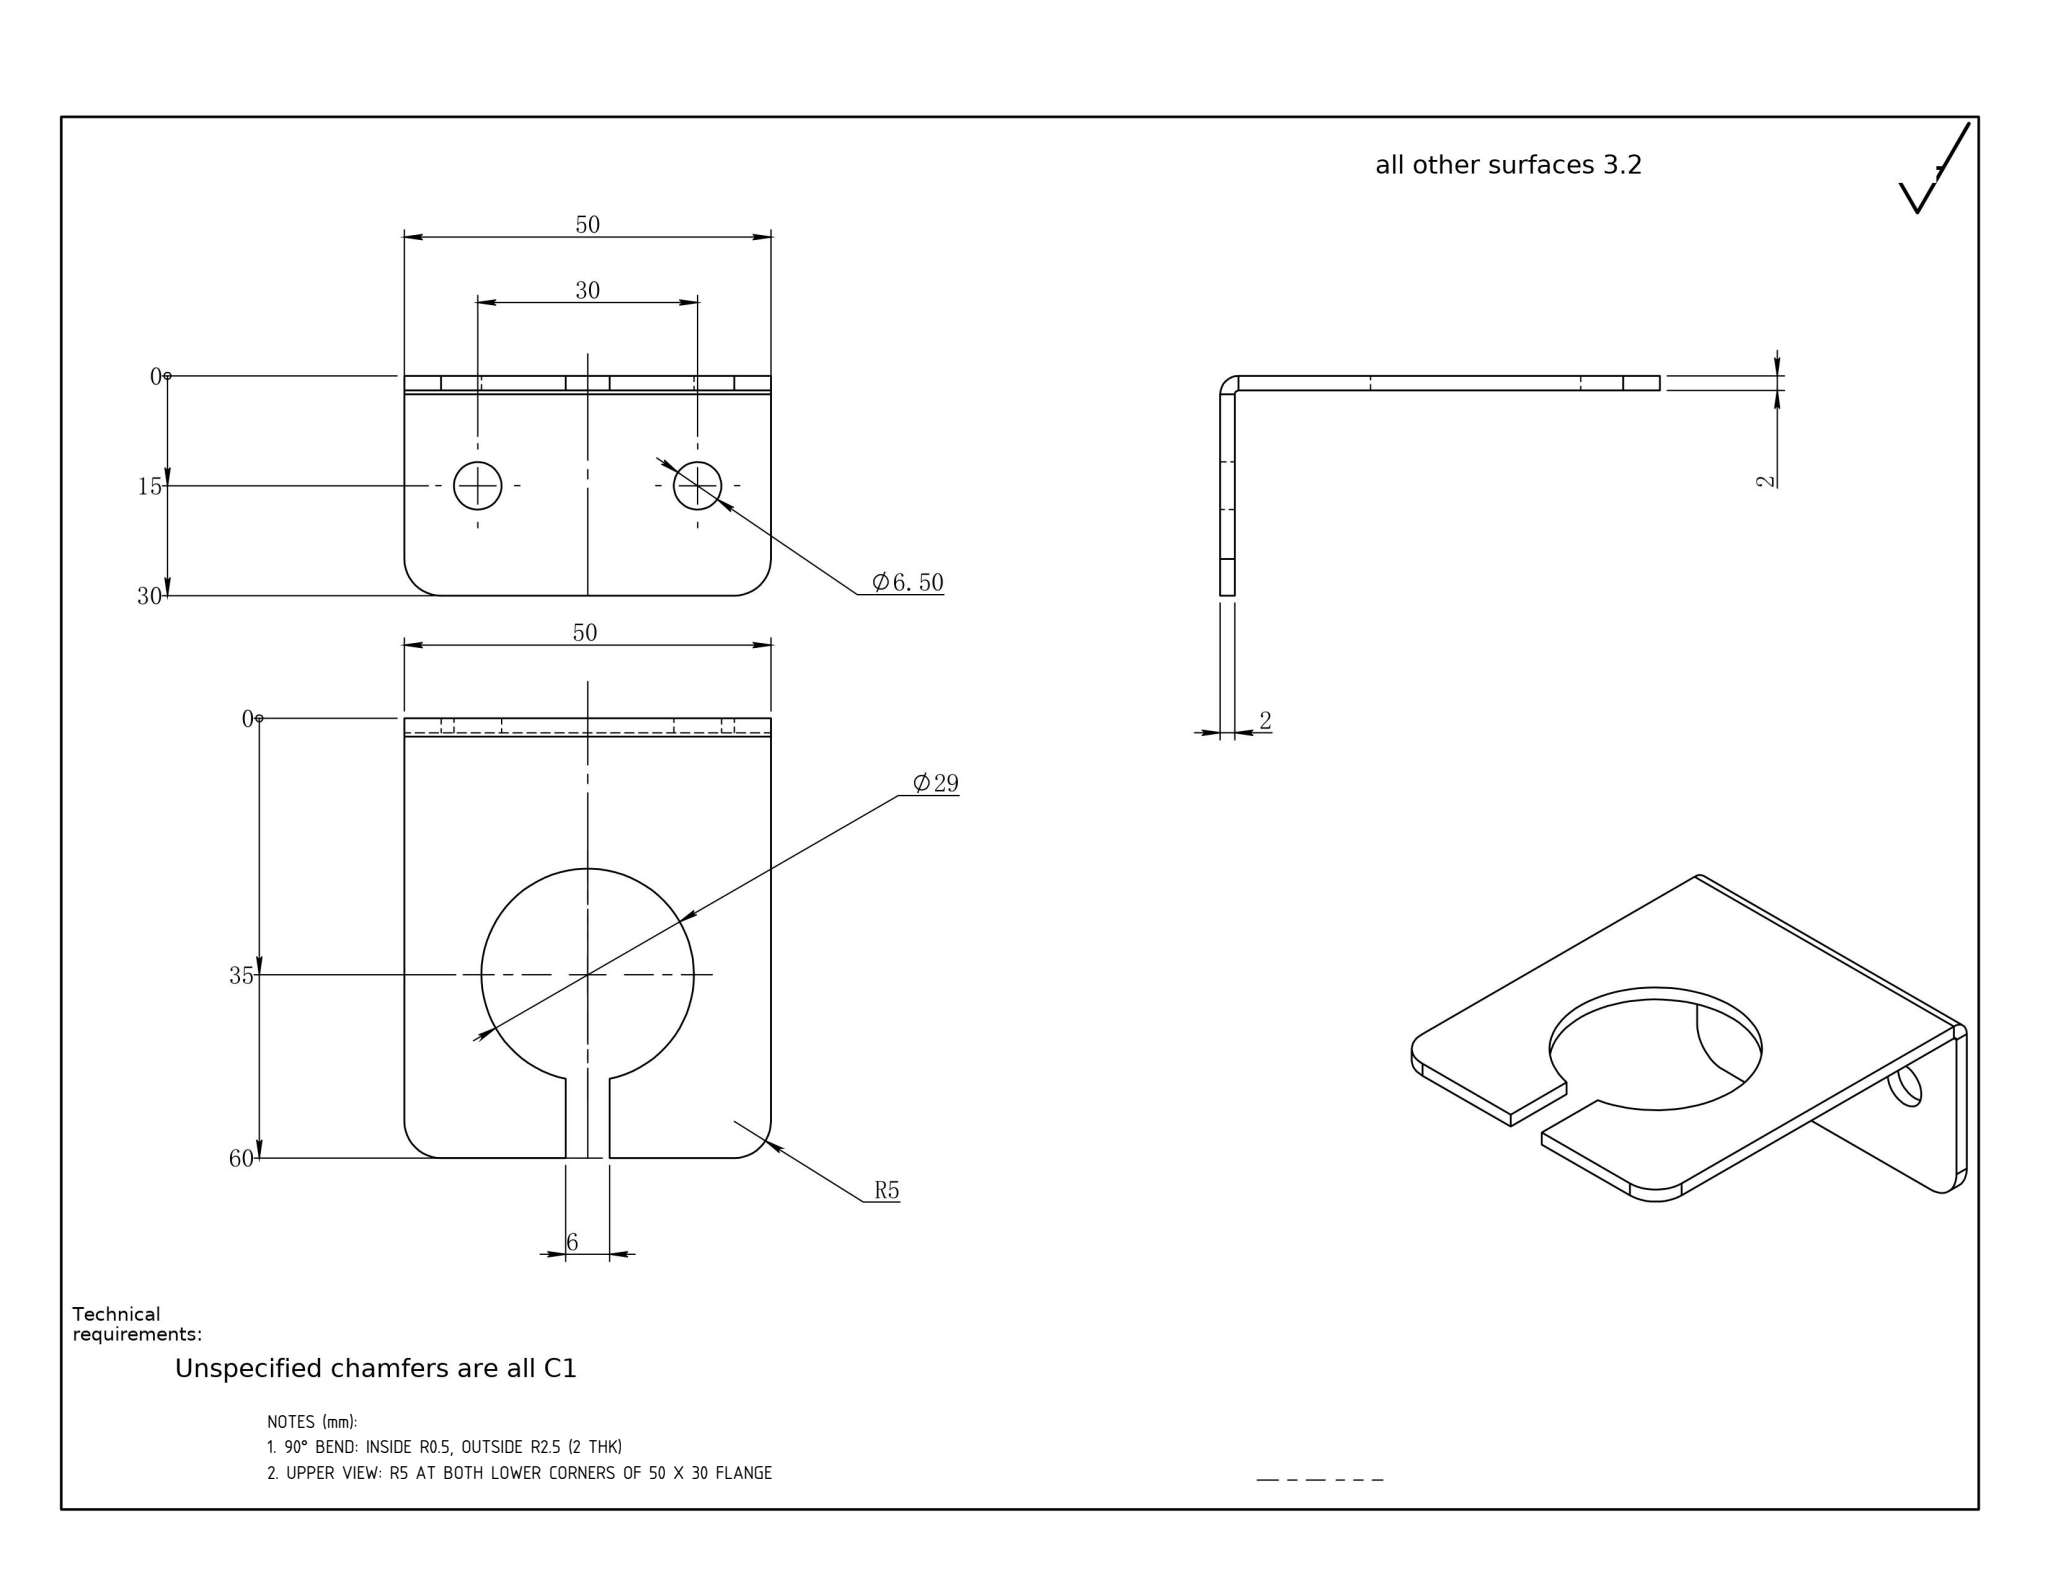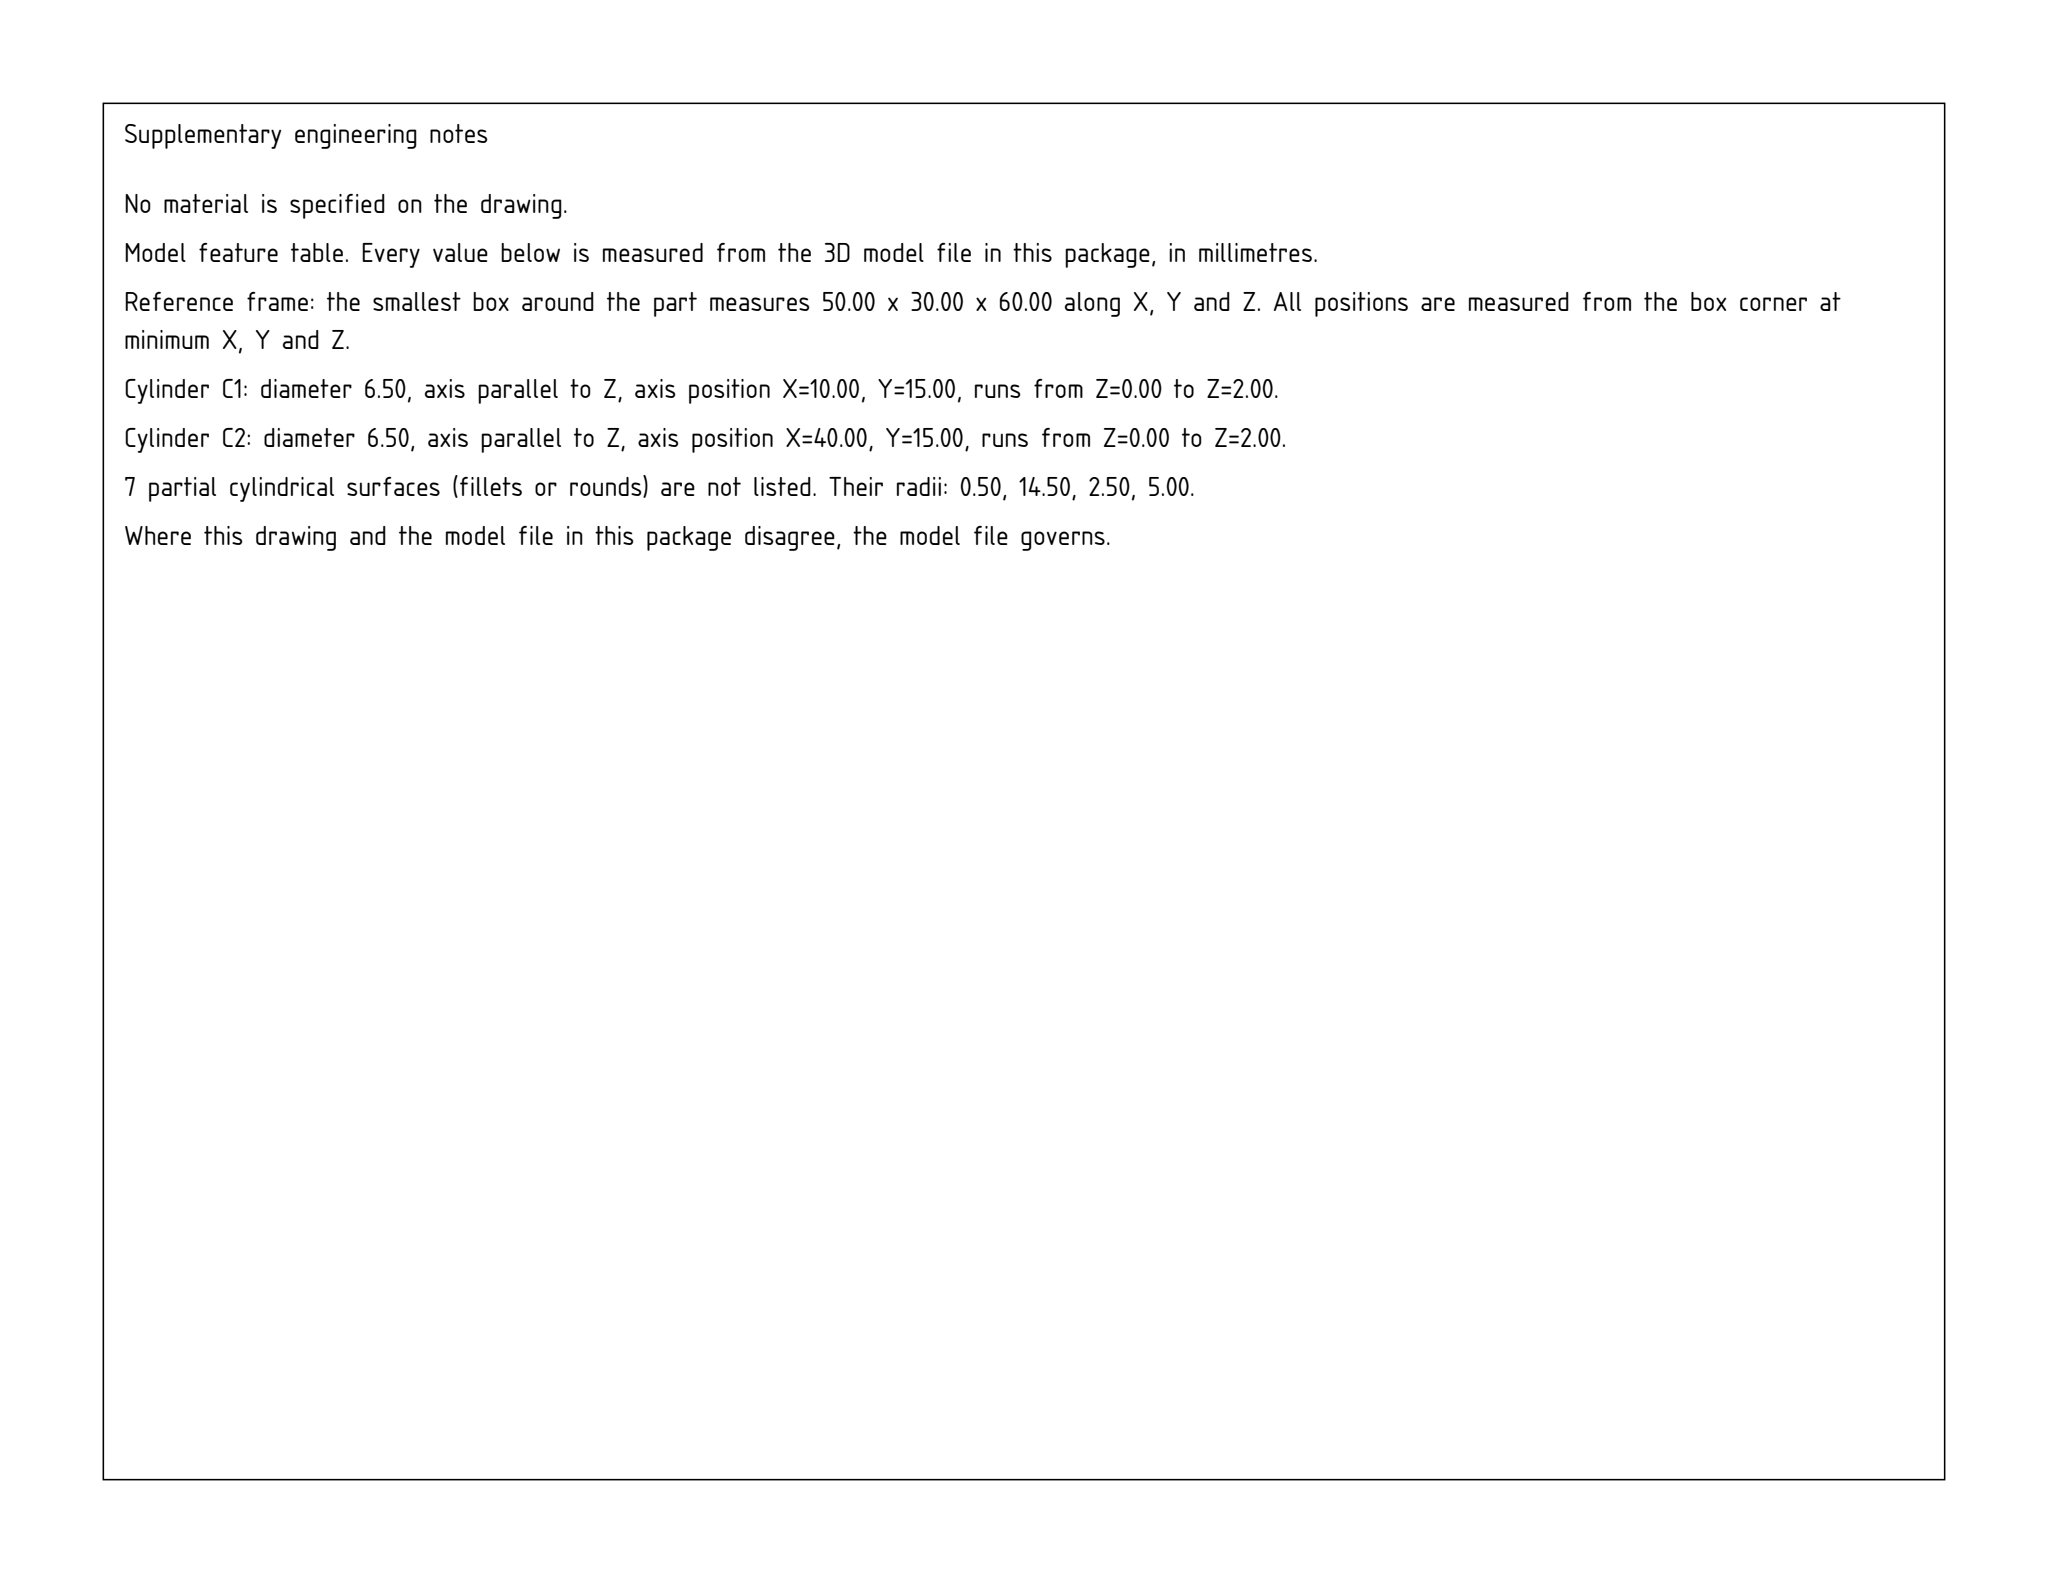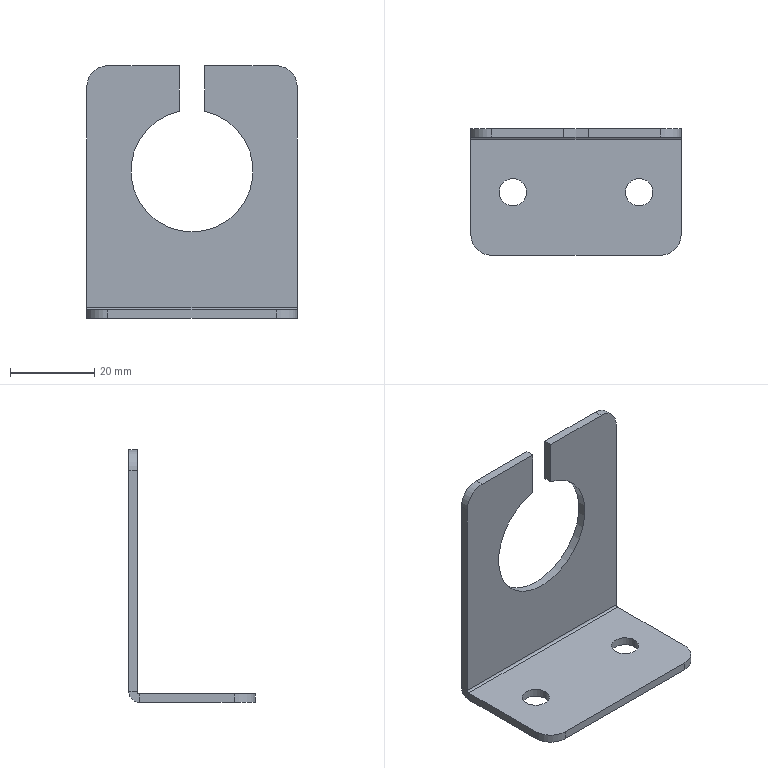Part | SolidWorks | mm | 1 solid | 26 faces | box 50 x 30 x 60 mm | volume 7112 mm3 | plane 15 | cylinder 11 | commonest cylinder face diameters 6.5 x4 10 x4 29 x1 5 x1 1 x1
Drawing notes:
90° BEND: INSIDE R0.5, OUTSIDE R2.5 (2 THK) | from the solid: cyl dia 1.0 & 5.0, axis x at y=27.5, z=2.5, len 50 = bend inner/outer radii with 2 wall
UPPER VIEW: R5 AT BOTH LOWER CORNERS OF 50 X 30 FLANGE | from the solid: Ø10 cyls, axis z, at (5,5) & (45,5), len 2 = R5 fillets on flange free edge (y=0 side), flange y 0-30, thk z 0-2
STEP:
#1=CARTESIAN_POINT('',(-18.25,-15.,-0.));
#2=VERTEX_POINT('',#1);
#3=CARTESIAN_POINT('',(-11.75,-15.,-0.));
#4=VERTEX_POINT('',#3);
#5=CARTESIAN_POINT('',(-15.,-15.,-0.));
#6=DIRECTION('',(0.,0.,1.));
#7=DIRECTION('',(1.,0.,0.));
#8=AXIS2_PLACEMENT_3D('',#5,#6,#7);
#9=CIRCLE('',#8,3.25);
#10=EDGE_CURVE('',#2,#4,#9,.T.);
#11=ORIENTED_EDGE('',*,*,#10,.F.);
#12=CARTESIAN_POINT('',(-18.25,-15.,2.));
#13=VERTEX_POINT('',#12);
#14=CARTESIAN_POINT('',(-18.25,-15.,2.));
#15=DIRECTION('',(0.,0.,1.));
#16=VECTOR('',#15,1000.);
#17=LINE('',#14,#16);
#18=EDGE_CURVE('',#2,#13,#17,.T.);
#19=ORIENTED_EDGE('',*,*,#18,.T.);
#20=CARTESIAN_POINT('',(-11.75,-15.,2.));
#21=VERTEX_POINT('',#20);
#22=CARTESIAN_POINT('',(-15.,-15.,2.));
#23=DIRECTION('',(0.,0.,1.));
#24=DIRECTION('',(1.,0.,0.));
#25=AXIS2_PLACEMENT_3D('',#22,#23,#24);
#26=CIRCLE('',#25,3.25);
#27=EDGE_CURVE('',#13,#21,#26,.T.);
#28=ORIENTED_EDGE('',*,*,#27,.T.);
#29=CARTESIAN_POINT('',(-11.75,-15.,2.));
#30=DIRECTION('',(0.,0.,1.));
#31=VECTOR('',#30,1000.);
#32=LINE('',#29,#31);
#33=EDGE_CURVE('',#4,#21,#32,.T.);
#34=ORIENTED_EDGE('',*,*,#33,.F.);
#35=EDGE_LOOP('',(#11,#19,#28,#34));
#36=FACE_OUTER_BOUND('',#35,.T.);
#37=CARTESIAN_POINT('',(-15.,-15.,2.));
#38=DIRECTION('',(0.,0.,1.));
#39=DIRECTION('',(1.,0.,0.));
#40=AXIS2_PLACEMENT_3D('',#37,#38,#39);
#41=CYLINDRICAL_SURFACE('',#40,3.25);
#42=ADVANCED_FACE('',(#36),#41,.F.);
#43=CARTESIAN_POINT('',(11.75,-15.,-0.));
#44=VERTEX_POINT('',#43);
#45=CARTESIAN_POINT('',(18.25,-15.,-0.));
#46=VERTEX_POINT('',#45);
#47=CARTESIAN_POINT('',(15.,-15.,-0.));
#48=DIRECTION('',(0.,0.,1.));
#49=DIRECTION('',(1.,0.,0.));
#50=AXIS2_PLACEMENT_3D('',#47,#48,#49);
#51=CIRCLE('',#50,3.25);
#52=EDGE_CURVE('',#44,#46,#51,.T.);
#53=ORIENTED_EDGE('',*,*,#52,.F.);
#54=CARTESIAN_POINT('',(11.75,-15.,2.));
#55=VERTEX_POINT('',#54);
#56=CARTESIAN_POINT('',(11.75,-15.,2.));
#57=DIRECTION('',(0.,0.,1.));
#58=VECTOR('',#57,1000.);
#59=LINE('',#56,#58);
#60=EDGE_CURVE('',#44,#55,#59,.T.);
#61=ORIENTED_EDGE('',*,*,#60,.T.);
#62=CARTESIAN_POINT('',(18.25,-15.,2.));
#63=VERTEX_POINT('',#62);
#64=CARTESIAN_POINT('',(15.,-15.,2.));
#65=DIRECTION('',(0.,0.,1.));
#66=DIRECTION('',(1.,0.,0.));
#67=AXIS2_PLACEMENT_3D('',#64,#65,#66);
#68=CIRCLE('',#67,3.25);
#69=EDGE_CURVE('',#55,#63,#68,.T.);
#70=ORIENTED_EDGE('',*,*,#69,.T.);
#71=CARTESIAN_POINT('',(18.25,-15.,2.));
#72=DIRECTION('',(0.,0.,1.));
#73=VECTOR('',#72,1000.);
#74=LINE('',#71,#73);
#75=EDGE_CURVE('',#46,#63,#74,.T.);
#76=ORIENTED_EDGE('',*,*,#75,.F.);
#77=EDGE_LOOP('',(#53,#61,#70,#76));
#78=FACE_OUTER_BOUND('',#77,.T.);
#79=CARTESIAN_POINT('',(15.,-15.,2.));
#80=DIRECTION('',(0.,0.,1.));
#81=DIRECTION('',(1.,0.,0.));
#82=AXIS2_PLACEMENT_3D('',#79,#80,#81);
#83=CYLINDRICAL_SURFACE('',#82,3.25);
#84=ADVANCED_FACE('',(#78),#83,.F.);
#85=CARTESIAN_POINT('',(3.,-0.,49.186));
#86=VERTEX_POINT('',#85);
#87=CARTESIAN_POINT('',(-3.,-0.,49.186));
#88=VERTEX_POINT('',#87);
#89=CARTESIAN_POINT('',(0.,-0.,35.));
#90=DIRECTION('',(0.,1.,0.));
#91=DIRECTION('',(0.,-0.,1.));
#92=AXIS2_PLACEMENT_3D('',#89,#90,#91);
#93=CIRCLE('',#92,14.5);
#94=EDGE_CURVE('',#86,#88,#93,.T.);
#95=ORIENTED_EDGE('',*,*,#94,.F.);
#96=CARTESIAN_POINT('',(3.,-0.,60.));
#97=VERTEX_POINT('',#96);
#98=CARTESIAN_POINT('',(3.,0.,0.));
#99=DIRECTION('',(0.,0.,-1.));
#100=VECTOR('',#99,1000.);
#101=LINE('',#98,#100);
#102=EDGE_CURVE('',#97,#86,#101,.T.);
#103=ORIENTED_EDGE('',*,*,#102,.F.);
#104=CARTESIAN_POINT('',(20.,-0.,60.));
#105=VERTEX_POINT('',#104);
#106=CARTESIAN_POINT('',(25.,-0.,60.));
#107=DIRECTION('',(-1.,0.,0.));
#108=VECTOR('',#107,1000.);
#109=LINE('',#106,#108);
#110=EDGE_CURVE('',#105,#97,#109,.T.);
#111=ORIENTED_EDGE('',*,*,#110,.F.);
#112=CARTESIAN_POINT('',(25.,-0.,55.));
#113=VERTEX_POINT('',#112);
#114=CARTESIAN_POINT('',(20.,-0.,55.));
#115=DIRECTION('',(0.,1.,0.));
#116=DIRECTION('',(0.,-0.,1.));
#117=AXIS2_PLACEMENT_3D('',#114,#115,#116);
#118=CIRCLE('',#117,5.);
#119=EDGE_CURVE('',#105,#113,#118,.T.);
#120=ORIENTED_EDGE('',*,*,#119,.T.);
#121=CARTESIAN_POINT('',(25.,-0.,2.5));
#122=VERTEX_POINT('',#121);
#123=CARTESIAN_POINT('',(25.,0.,0.));
#124=DIRECTION('',(0.,0.,-1.));
#125=VECTOR('',#124,1000.);
#126=LINE('',#123,#125);
#127=EDGE_CURVE('',#113,#122,#126,.T.);
#128=ORIENTED_EDGE('',*,*,#127,.T.);
#129=CARTESIAN_POINT('',(-25.,-0.,2.5));
#130=VERTEX_POINT('',#129);
#131=CARTESIAN_POINT('',(25.,-0.,2.5));
#132=DIRECTION('',(-1.,0.,0.));
#133=VECTOR('',#132,1000.);
#134=LINE('',#131,#133);
#135=EDGE_CURVE('',#122,#130,#134,.T.);
#136=ORIENTED_EDGE('',*,*,#135,.T.);
#137=CARTESIAN_POINT('',(-25.,-0.,55.));
#138=VERTEX_POINT('',#137);
#139=CARTESIAN_POINT('',(-25.,0.,0.));
#140=DIRECTION('',(0.,0.,-1.));
#141=VECTOR('',#140,1000.);
#142=LINE('',#139,#141);
#143=EDGE_CURVE('',#138,#130,#142,.T.);
#144=ORIENTED_EDGE('',*,*,#143,.F.);
#145=CARTESIAN_POINT('',(-20.,-0.,60.));
#146=VERTEX_POINT('',#145);
#147=CARTESIAN_POINT('',(-20.,-0.,55.));
#148=DIRECTION('',(0.,1.,0.));
#149=DIRECTION('',(0.,-0.,1.));
#150=AXIS2_PLACEMENT_3D('',#147,#148,#149);
#151=CIRCLE('',#150,5.);
#152=EDGE_CURVE('',#138,#146,#151,.T.);
#153=ORIENTED_EDGE('',*,*,#152,.T.);
#154=CARTESIAN_POINT('',(-3.,-0.,60.));
#155=VERTEX_POINT('',#154);
#156=CARTESIAN_POINT('',(25.,-0.,60.));
#157=DIRECTION('',(-1.,0.,0.));
#158=VECTOR('',#157,1000.);
#159=LINE('',#156,#158);
#160=EDGE_CURVE('',#155,#146,#159,.T.);
#161=ORIENTED_EDGE('',*,*,#160,.F.);
#162=CARTESIAN_POINT('',(-3.,0.,0.));
#163=DIRECTION('',(0.,-0.,1.));
#164=VECTOR('',#163,1000.);
#165=LINE('',#162,#164);
#166=EDGE_CURVE('',#88,#155,#165,.T.);
#167=ORIENTED_EDGE('',*,*,#166,.F.);
#168=EDGE_LOOP('',(#95,#103,#111,#120,#128,#136,#144,#153,#161,#167));
#169=FACE_OUTER_BOUND('',#168,.T.);
#170=CARTESIAN_POINT('',(25.,0.,0.));
#171=DIRECTION('',(0.,1.,0.));
#172=DIRECTION('',(0.,-0.,1.));
#173=AXIS2_PLACEMENT_3D('',#170,#171,#172);
#174=PLANE('',#173);
#175=ADVANCED_FACE('',(#169),#174,.T.);
#176=ORIENTED_EDGE('',*,*,#110,.T.);
#177=CARTESIAN_POINT('',(3.,-2.,60.));
#178=VERTEX_POINT('',#177);
#179=CARTESIAN_POINT('',(3.,-2.,60.));
#180=DIRECTION('',(0.,1.,0.));
#181=VECTOR('',#180,1000.);
#182=LINE('',#179,#181);
#183=EDGE_CURVE('',#178,#97,#182,.T.);
#184=ORIENTED_EDGE('',*,*,#183,.F.);
#185=CARTESIAN_POINT('',(20.,-2.,60.));
#186=VERTEX_POINT('',#185);
#187=CARTESIAN_POINT('',(25.,-2.,60.));
#188=DIRECTION('',(-1.,0.,0.));
#189=VECTOR('',#188,1000.);
#190=LINE('',#187,#189);
#191=EDGE_CURVE('',#186,#178,#190,.T.);
#192=ORIENTED_EDGE('',*,*,#191,.F.);
#193=CARTESIAN_POINT('',(20.,-2.,60.));
#194=DIRECTION('',(0.,1.,0.));
#195=VECTOR('',#194,1000.);
#196=LINE('',#193,#195);
#197=EDGE_CURVE('',#186,#105,#196,.T.);
#198=ORIENTED_EDGE('',*,*,#197,.T.);
#199=EDGE_LOOP('',(#176,#184,#192,#198));
#200=FACE_OUTER_BOUND('',#199,.T.);
#201=CARTESIAN_POINT('',(25.,-2.,60.));
#202=DIRECTION('',(0.,0.,1.));
#203=DIRECTION('',(1.,0.,0.));
#204=AXIS2_PLACEMENT_3D('',#201,#202,#203);
#205=PLANE('',#204);
#206=ADVANCED_FACE('',(#200),#205,.T.);
#207=CARTESIAN_POINT('',(-3.,-2.,60.));
#208=VERTEX_POINT('',#207);
#209=CARTESIAN_POINT('',(-20.,-2.,60.));
#210=VERTEX_POINT('',#209);
#211=CARTESIAN_POINT('',(25.,-2.,60.));
#212=DIRECTION('',(-1.,0.,0.));
#213=VECTOR('',#212,1000.);
#214=LINE('',#211,#213);
#215=EDGE_CURVE('',#208,#210,#214,.T.);
#216=ORIENTED_EDGE('',*,*,#215,.F.);
#217=CARTESIAN_POINT('',(-3.,-2.,60.));
#218=DIRECTION('',(0.,1.,0.));
#219=VECTOR('',#218,1000.);
#220=LINE('',#217,#219);
#221=EDGE_CURVE('',#208,#155,#220,.T.);
#222=ORIENTED_EDGE('',*,*,#221,.T.);
#223=ORIENTED_EDGE('',*,*,#160,.T.);
#224=CARTESIAN_POINT('',(-20.,-2.,60.));
#225=DIRECTION('',(0.,-1.,0.));
#226=VECTOR('',#225,1000.);
#227=LINE('',#224,#226);
#228=EDGE_CURVE('',#146,#210,#227,.T.);
#229=ORIENTED_EDGE('',*,*,#228,.T.);
#230=EDGE_LOOP('',(#216,#222,#223,#229));
#231=FACE_OUTER_BOUND('',#230,.T.);
#232=CARTESIAN_POINT('',(25.,-2.,60.));
#233=DIRECTION('',(0.,0.,1.));
#234=DIRECTION('',(1.,0.,0.));
#235=AXIS2_PLACEMENT_3D('',#232,#233,#234);
#236=PLANE('',#235);
#237=ADVANCED_FACE('',(#231),#236,.T.);
#238=CARTESIAN_POINT('',(3.,-2.,49.186));
#239=VERTEX_POINT('',#238);
#240=CARTESIAN_POINT('',(3.,-2.,-0.));
#241=DIRECTION('',(0.,0.,-1.));
#242=VECTOR('',#241,1000.);
#243=LINE('',#240,#242);
#244=EDGE_CURVE('',#178,#239,#243,.T.);
#245=ORIENTED_EDGE('',*,*,#244,.T.);
#246=CARTESIAN_POINT('',(-3.,-2.,49.186));
#247=VERTEX_POINT('',#246);
#248=CARTESIAN_POINT('',(0.,-2.,35.));
#249=DIRECTION('',(0.,1.,0.));
#250=DIRECTION('',(0.,-0.,1.));
#251=AXIS2_PLACEMENT_3D('',#248,#249,#250);
#252=CIRCLE('',#251,14.5);
#253=EDGE_CURVE('',#239,#247,#252,.T.);
#254=ORIENTED_EDGE('',*,*,#253,.T.);
#255=CARTESIAN_POINT('',(-3.,-2.,-0.));
#256=DIRECTION('',(0.,-0.,1.));
#257=VECTOR('',#256,1000.);
#258=LINE('',#255,#257);
#259=EDGE_CURVE('',#247,#208,#258,.T.);
#260=ORIENTED_EDGE('',*,*,#259,.T.);
#261=ORIENTED_EDGE('',*,*,#215,.T.);
#262=CARTESIAN_POINT('',(-25.,-2.,55.));
#263=VERTEX_POINT('',#262);
#264=CARTESIAN_POINT('',(-20.,-2.,55.));
#265=DIRECTION('',(0.,-1.,-0.));
#266=DIRECTION('',(0.,-0.,1.));
#267=AXIS2_PLACEMENT_3D('',#264,#265,#266);
#268=CIRCLE('',#267,5.);
#269=EDGE_CURVE('',#210,#263,#268,.T.);
#270=ORIENTED_EDGE('',*,*,#269,.T.);
#271=CARTESIAN_POINT('',(-25.,-2.,2.5));
#272=VERTEX_POINT('',#271);
#273=CARTESIAN_POINT('',(-25.,-2.,-0.));
#274=DIRECTION('',(0.,0.,-1.));
#275=VECTOR('',#274,1000.);
#276=LINE('',#273,#275);
#277=EDGE_CURVE('',#263,#272,#276,.T.);
#278=ORIENTED_EDGE('',*,*,#277,.T.);
#279=CARTESIAN_POINT('',(25.,-2.,2.5));
#280=VERTEX_POINT('',#279);
#281=CARTESIAN_POINT('',(25.,-2.,2.5));
#282=DIRECTION('',(-1.,0.,0.));
#283=VECTOR('',#282,1000.);
#284=LINE('',#281,#283);
#285=EDGE_CURVE('',#280,#272,#284,.T.);
#286=ORIENTED_EDGE('',*,*,#285,.F.);
#287=CARTESIAN_POINT('',(25.,-2.,55.));
#288=VERTEX_POINT('',#287);
#289=CARTESIAN_POINT('',(25.,-2.,-0.));
#290=DIRECTION('',(0.,0.,-1.));
#291=VECTOR('',#290,1000.);
#292=LINE('',#289,#291);
#293=EDGE_CURVE('',#288,#280,#292,.T.);
#294=ORIENTED_EDGE('',*,*,#293,.F.);
#295=CARTESIAN_POINT('',(20.,-2.,55.));
#296=DIRECTION('',(0.,-1.,-0.));
#297=DIRECTION('',(0.,-0.,1.));
#298=AXIS2_PLACEMENT_3D('',#295,#296,#297);
#299=CIRCLE('',#298,5.);
#300=EDGE_CURVE('',#288,#186,#299,.T.);
#301=ORIENTED_EDGE('',*,*,#300,.T.);
#302=ORIENTED_EDGE('',*,*,#191,.T.);
#303=EDGE_LOOP('',(#245,#254,#260,#261,#270,#278,#286,#294,#301,#302));
#304=FACE_OUTER_BOUND('',#303,.T.);
#305=CARTESIAN_POINT('',(25.,-2.,-0.));
#306=DIRECTION('',(0.,1.,0.));
#307=DIRECTION('',(0.,-0.,1.));
#308=AXIS2_PLACEMENT_3D('',#305,#306,#307);
#309=PLANE('',#308);
#310=ADVANCED_FACE('',(#304),#309,.F.);
#311=CARTESIAN_POINT('',(3.,-2.,49.186));
#312=DIRECTION('',(0.,1.,0.));
#313=VECTOR('',#312,1000.);
#314=LINE('',#311,#313);
#315=EDGE_CURVE('',#239,#86,#314,.T.);
#316=ORIENTED_EDGE('',*,*,#315,.T.);
#317=ORIENTED_EDGE('',*,*,#94,.T.);
#318=CARTESIAN_POINT('',(-3.,-2.,49.186));
#319=DIRECTION('',(0.,1.,0.));
#320=VECTOR('',#319,1000.);
#321=LINE('',#318,#320);
#322=EDGE_CURVE('',#247,#88,#321,.T.);
#323=ORIENTED_EDGE('',*,*,#322,.F.);
#324=ORIENTED_EDGE('',*,*,#253,.F.);
#325=EDGE_LOOP('',(#316,#317,#323,#324));
#326=FACE_OUTER_BOUND('',#325,.T.);
#327=CARTESIAN_POINT('',(0.,-30.,35.));
#328=DIRECTION('',(0.,1.,0.));
#329=DIRECTION('',(0.,-0.,1.));
#330=AXIS2_PLACEMENT_3D('',#327,#328,#329);
#331=CYLINDRICAL_SURFACE('',#330,14.5);
#332=ADVANCED_FACE('',(#326),#331,.F.);
#333=CARTESIAN_POINT('',(25.,-2.5,-0.));
#334=VERTEX_POINT('',#333);
#335=CARTESIAN_POINT('',(25.,-2.5,2.));
#336=VERTEX_POINT('',#335);
#337=CARTESIAN_POINT('',(25.,-2.5,-0.));
#338=DIRECTION('',(0.,-0.,1.));
#339=VECTOR('',#338,1000.);
#340=LINE('',#337,#339);
#341=EDGE_CURVE('',#334,#336,#340,.T.);
#342=ORIENTED_EDGE('',*,*,#341,.F.);
#343=CARTESIAN_POINT('',(25.,-2.5,2.5));
#344=DIRECTION('',(-1.,0.,0.));
#345=DIRECTION('',(0.,0.,-1.));
#346=AXIS2_PLACEMENT_3D('',#343,#344,#345);
#347=CIRCLE('',#346,2.5);
#348=EDGE_CURVE('',#122,#334,#347,.T.);
#349=ORIENTED_EDGE('',*,*,#348,.F.);
#350=CARTESIAN_POINT('',(25.,-2.,2.5));
#351=DIRECTION('',(0.,1.,0.));
#352=VECTOR('',#351,1000.);
#353=LINE('',#350,#352);
#354=EDGE_CURVE('',#280,#122,#353,.T.);
#355=ORIENTED_EDGE('',*,*,#354,.F.);
#356=CARTESIAN_POINT('',(25.,-2.5,2.5));
#357=DIRECTION('',(-1.,0.,0.));
#358=DIRECTION('',(0.,0.,-1.));
#359=AXIS2_PLACEMENT_3D('',#356,#357,#358);
#360=CIRCLE('',#359,0.5);
#361=EDGE_CURVE('',#280,#336,#360,.T.);
#362=ORIENTED_EDGE('',*,*,#361,.T.);
#363=EDGE_LOOP('',(#342,#349,#355,#362));
#364=FACE_OUTER_BOUND('',#363,.T.);
#365=CARTESIAN_POINT('',(25.,-2.5,-0.));
#366=DIRECTION('',(1.,0.,0.));
#367=DIRECTION('',(0.,0.,-1.));
#368=AXIS2_PLACEMENT_3D('',#365,#366,#367);
#369=PLANE('',#368);
#370=ADVANCED_FACE('',(#364),#369,.T.);
#371=CARTESIAN_POINT('',(25.,-25.,2.));
#372=VERTEX_POINT('',#371);
#373=CARTESIAN_POINT('',(25.,-0.,2.));
#374=DIRECTION('',(0.,-1.,-0.));
#375=VECTOR('',#374,1000.);
#376=LINE('',#373,#375);
#377=EDGE_CURVE('',#336,#372,#376,.T.);
#378=ORIENTED_EDGE('',*,*,#377,.T.);
#379=CARTESIAN_POINT('',(25.,-25.,-0.));
#380=VERTEX_POINT('',#379);
#381=CARTESIAN_POINT('',(25.,-25.,2.5));
#382=DIRECTION('',(0.,0.,-1.));
#383=VECTOR('',#382,1000.);
#384=LINE('',#381,#383);
#385=EDGE_CURVE('',#372,#380,#384,.T.);
#386=ORIENTED_EDGE('',*,*,#385,.T.);
#387=CARTESIAN_POINT('',(25.,0.,0.));
#388=DIRECTION('',(0.,-1.,-0.));
#389=VECTOR('',#388,1000.);
#390=LINE('',#387,#389);
#391=EDGE_CURVE('',#334,#380,#390,.T.);
#392=ORIENTED_EDGE('',*,*,#391,.F.);
#393=ORIENTED_EDGE('',*,*,#341,.T.);
#394=EDGE_LOOP('',(#378,#386,#392,#393));
#395=FACE_OUTER_BOUND('',#394,.T.);
#396=CARTESIAN_POINT('',(25.,-2.,2.5));
#397=DIRECTION('',(1.,0.,0.));
#398=DIRECTION('',(0.,0.,-1.));
#399=AXIS2_PLACEMENT_3D('',#396,#397,#398);
#400=PLANE('',#399);
#401=ADVANCED_FACE('',(#395),#400,.T.);
#402=CARTESIAN_POINT('',(-25.,-0.,2.5));
#403=DIRECTION('',(0.,-1.,-0.));
#404=VECTOR('',#403,1000.);
#405=LINE('',#402,#404);
#406=EDGE_CURVE('',#130,#272,#405,.T.);
#407=ORIENTED_EDGE('',*,*,#406,.F.);
#408=CARTESIAN_POINT('',(-25.,-2.5,-0.));
#409=VERTEX_POINT('',#408);
#410=CARTESIAN_POINT('',(-25.,-2.5,2.5));
#411=DIRECTION('',(-1.,0.,0.));
#412=DIRECTION('',(0.,0.,-1.));
#413=AXIS2_PLACEMENT_3D('',#410,#411,#412);
#414=CIRCLE('',#413,2.5);
#415=EDGE_CURVE('',#130,#409,#414,.T.);
#416=ORIENTED_EDGE('',*,*,#415,.T.);
#417=CARTESIAN_POINT('',(-25.,-2.5,2.));
#418=VERTEX_POINT('',#417);
#419=CARTESIAN_POINT('',(-25.,-2.5,2.));
#420=DIRECTION('',(0.,0.,-1.));
#421=VECTOR('',#420,1000.);
#422=LINE('',#419,#421);
#423=EDGE_CURVE('',#418,#409,#422,.T.);
#424=ORIENTED_EDGE('',*,*,#423,.F.);
#425=CARTESIAN_POINT('',(-25.,-2.5,2.5));
#426=DIRECTION('',(-1.,0.,0.));
#427=DIRECTION('',(0.,0.,-1.));
#428=AXIS2_PLACEMENT_3D('',#425,#426,#427);
#429=CIRCLE('',#428,0.5);
#430=EDGE_CURVE('',#272,#418,#429,.T.);
#431=ORIENTED_EDGE('',*,*,#430,.F.);
#432=EDGE_LOOP('',(#407,#416,#424,#431));
#433=FACE_OUTER_BOUND('',#432,.T.);
#434=CARTESIAN_POINT('',(-25.,-0.,2.5));
#435=DIRECTION('',(-1.,0.,0.));
#436=DIRECTION('',(0.,0.,1.));
#437=AXIS2_PLACEMENT_3D('',#434,#435,#436);
#438=PLANE('',#437);
#439=ADVANCED_FACE('',(#433),#438,.T.);
#440=ORIENTED_EDGE('',*,*,#277,.F.);
#441=CARTESIAN_POINT('',(-25.,-2.5,55.));
#442=DIRECTION('',(0.,1.,0.));
#443=VECTOR('',#442,1000.);
#444=LINE('',#441,#443);
#445=EDGE_CURVE('',#263,#138,#444,.T.);
#446=ORIENTED_EDGE('',*,*,#445,.T.);
#447=ORIENTED_EDGE('',*,*,#143,.T.);
#448=ORIENTED_EDGE('',*,*,#406,.T.);
#449=EDGE_LOOP('',(#440,#446,#447,#448));
#450=FACE_OUTER_BOUND('',#449,.T.);
#451=CARTESIAN_POINT('',(-25.,-2.5,2.));
#452=DIRECTION('',(-1.,0.,0.));
#453=DIRECTION('',(0.,0.,1.));
#454=AXIS2_PLACEMENT_3D('',#451,#452,#453);
#455=PLANE('',#454);
#456=ADVANCED_FACE('',(#450),#455,.T.);
#457=CARTESIAN_POINT('',(-15.,-15.,2.));
#458=DIRECTION('',(0.,0.,1.));
#459=DIRECTION('',(1.,0.,0.));
#460=AXIS2_PLACEMENT_3D('',#457,#458,#459);
#461=CIRCLE('',#460,3.25);
#462=EDGE_CURVE('',#21,#13,#461,.T.);
#463=ORIENTED_EDGE('',*,*,#462,.F.);
#464=ORIENTED_EDGE('',*,*,#27,.F.);
#465=EDGE_LOOP('',(#463,#464));
#466=FACE_BOUND('',#465,.T.);
#467=CARTESIAN_POINT('',(15.,-15.,2.));
#468=DIRECTION('',(0.,0.,1.));
#469=DIRECTION('',(1.,0.,0.));
#470=AXIS2_PLACEMENT_3D('',#467,#468,#469);
#471=CIRCLE('',#470,3.25);
#472=EDGE_CURVE('',#63,#55,#471,.T.);
#473=ORIENTED_EDGE('',*,*,#472,.F.);
#474=ORIENTED_EDGE('',*,*,#69,.F.);
#475=EDGE_LOOP('',(#473,#474));
#476=FACE_BOUND('',#475,.T.);
#477=CARTESIAN_POINT('',(20.,-30.,2.));
#478=VERTEX_POINT('',#477);
#479=CARTESIAN_POINT('',(-20.,-30.,2.));
#480=VERTEX_POINT('',#479);
#481=CARTESIAN_POINT('',(25.,-30.,2.));
#482=DIRECTION('',(-1.,0.,0.));
#483=VECTOR('',#482,1000.);
#484=LINE('',#481,#483);
#485=EDGE_CURVE('',#478,#480,#484,.T.);
#486=ORIENTED_EDGE('',*,*,#485,.F.);
#487=CARTESIAN_POINT('',(20.,-25.,2.));
#488=DIRECTION('',(0.,-0.,1.));
#489=DIRECTION('',(0.,1.,0.));
#490=AXIS2_PLACEMENT_3D('',#487,#488,#489);
#491=CIRCLE('',#490,5.);
#492=EDGE_CURVE('',#478,#372,#491,.T.);
#493=ORIENTED_EDGE('',*,*,#492,.T.);
#494=ORIENTED_EDGE('',*,*,#377,.F.);
#495=CARTESIAN_POINT('',(25.,-2.5,2.));
#496=DIRECTION('',(-1.,0.,0.));
#497=VECTOR('',#496,1000.);
#498=LINE('',#495,#497);
#499=EDGE_CURVE('',#336,#418,#498,.T.);
#500=ORIENTED_EDGE('',*,*,#499,.T.);
#501=CARTESIAN_POINT('',(-25.,-25.,2.));
#502=VERTEX_POINT('',#501);
#503=CARTESIAN_POINT('',(-25.,-0.,2.));
#504=DIRECTION('',(0.,-1.,-0.));
#505=VECTOR('',#504,1000.);
#506=LINE('',#503,#505);
#507=EDGE_CURVE('',#418,#502,#506,.T.);
#508=ORIENTED_EDGE('',*,*,#507,.T.);
#509=CARTESIAN_POINT('',(-20.,-25.,2.));
#510=DIRECTION('',(0.,-0.,1.));
#511=DIRECTION('',(0.,1.,0.));
#512=AXIS2_PLACEMENT_3D('',#509,#510,#511);
#513=CIRCLE('',#512,5.);
#514=EDGE_CURVE('',#502,#480,#513,.T.);
#515=ORIENTED_EDGE('',*,*,#514,.T.);
#516=EDGE_LOOP('',(#486,#493,#494,#500,#508,#515));
#517=FACE_OUTER_BOUND('',#516,.T.);
#518=CARTESIAN_POINT('',(25.,-0.,2.));
#519=DIRECTION('',(0.,0.,-1.));
#520=DIRECTION('',(0.,1.,0.));
#521=AXIS2_PLACEMENT_3D('',#518,#519,#520);
#522=PLANE('',#521);
#523=ADVANCED_FACE('',(#466,#476,#517),#522,.F.);
#524=CARTESIAN_POINT('',(20.,-30.,-0.));
#525=VERTEX_POINT('',#524);
#526=CARTESIAN_POINT('',(-20.,-30.,-0.));
#527=VERTEX_POINT('',#526);
#528=CARTESIAN_POINT('',(25.,-30.,-0.));
#529=DIRECTION('',(-1.,0.,0.));
#530=VECTOR('',#529,1000.);
#531=LINE('',#528,#530);
#532=EDGE_CURVE('',#525,#527,#531,.T.);
#533=ORIENTED_EDGE('',*,*,#532,.F.);
#534=CARTESIAN_POINT('',(20.,-30.,-0.));
#535=DIRECTION('',(0.,0.,1.));
#536=VECTOR('',#535,1000.);
#537=LINE('',#534,#536);
#538=EDGE_CURVE('',#525,#478,#537,.T.);
#539=ORIENTED_EDGE('',*,*,#538,.T.);
#540=ORIENTED_EDGE('',*,*,#485,.T.);
#541=CARTESIAN_POINT('',(-20.,-30.,-0.));
#542=DIRECTION('',(0.,0.,-1.));
#543=VECTOR('',#542,1000.);
#544=LINE('',#541,#543);
#545=EDGE_CURVE('',#480,#527,#544,.T.);
#546=ORIENTED_EDGE('',*,*,#545,.T.);
#547=EDGE_LOOP('',(#533,#539,#540,#546));
#548=FACE_OUTER_BOUND('',#547,.T.);
#549=CARTESIAN_POINT('',(25.,-30.,-0.));
#550=DIRECTION('',(0.,-1.,0.));
#551=DIRECTION('',(0.,0.,-1.));
#552=AXIS2_PLACEMENT_3D('',#549,#550,#551);
#553=PLANE('',#552);
#554=ADVANCED_FACE('',(#548),#553,.T.);
#555=CARTESIAN_POINT('',(-15.,-15.,-0.));
#556=DIRECTION('',(0.,0.,1.));
#557=DIRECTION('',(1.,0.,0.));
#558=AXIS2_PLACEMENT_3D('',#555,#556,#557);
#559=CIRCLE('',#558,3.25);
#560=EDGE_CURVE('',#4,#2,#559,.T.);
#561=ORIENTED_EDGE('',*,*,#560,.T.);
#562=ORIENTED_EDGE('',*,*,#10,.T.);
#563=EDGE_LOOP('',(#561,#562));
#564=FACE_BOUND('',#563,.T.);
#565=CARTESIAN_POINT('',(15.,-15.,-0.));
#566=DIRECTION('',(0.,0.,1.));
#567=DIRECTION('',(1.,0.,0.));
#568=AXIS2_PLACEMENT_3D('',#565,#566,#567);
#569=CIRCLE('',#568,3.25);
#570=EDGE_CURVE('',#46,#44,#569,.T.);
#571=ORIENTED_EDGE('',*,*,#570,.T.);
#572=ORIENTED_EDGE('',*,*,#52,.T.);
#573=EDGE_LOOP('',(#571,#572));
#574=FACE_BOUND('',#573,.T.);
#575=ORIENTED_EDGE('',*,*,#391,.T.);
#576=CARTESIAN_POINT('',(20.,-25.,-0.));
#577=DIRECTION('',(0.,0.,-1.));
#578=DIRECTION('',(0.,1.,0.));
#579=AXIS2_PLACEMENT_3D('',#576,#577,#578);
#580=CIRCLE('',#579,5.);
#581=EDGE_CURVE('',#380,#525,#580,.T.);
#582=ORIENTED_EDGE('',*,*,#581,.T.);
#583=ORIENTED_EDGE('',*,*,#532,.T.);
#584=CARTESIAN_POINT('',(-25.,-25.,-0.));
#585=VERTEX_POINT('',#584);
#586=CARTESIAN_POINT('',(-20.,-25.,-0.));
#587=DIRECTION('',(0.,0.,-1.));
#588=DIRECTION('',(0.,1.,0.));
#589=AXIS2_PLACEMENT_3D('',#586,#587,#588);
#590=CIRCLE('',#589,5.);
#591=EDGE_CURVE('',#527,#585,#590,.T.);
#592=ORIENTED_EDGE('',*,*,#591,.T.);
#593=CARTESIAN_POINT('',(-25.,0.,0.));
#594=DIRECTION('',(0.,-1.,-0.));
#595=VECTOR('',#594,1000.);
#596=LINE('',#593,#595);
#597=EDGE_CURVE('',#409,#585,#596,.T.);
#598=ORIENTED_EDGE('',*,*,#597,.F.);
#599=CARTESIAN_POINT('',(25.,-2.5,-0.));
#600=DIRECTION('',(-1.,0.,0.));
#601=VECTOR('',#600,1000.);
#602=LINE('',#599,#601);
#603=EDGE_CURVE('',#334,#409,#602,.T.);
#604=ORIENTED_EDGE('',*,*,#603,.F.);
#605=EDGE_LOOP('',(#575,#582,#583,#592,#598,#604));
#606=FACE_OUTER_BOUND('',#605,.T.);
#607=CARTESIAN_POINT('',(25.,0.,0.));
#608=DIRECTION('',(0.,0.,-1.));
#609=DIRECTION('',(0.,1.,0.));
#610=AXIS2_PLACEMENT_3D('',#607,#608,#609);
#611=PLANE('',#610);
#612=ADVANCED_FACE('',(#564,#574,#606),#611,.T.);
#613=ORIENTED_EDGE('',*,*,#415,.F.);
#614=ORIENTED_EDGE('',*,*,#135,.F.);
#615=ORIENTED_EDGE('',*,*,#348,.T.);
#616=ORIENTED_EDGE('',*,*,#603,.T.);
#617=EDGE_LOOP('',(#613,#614,#615,#616));
#618=FACE_OUTER_BOUND('',#617,.T.);
#619=CARTESIAN_POINT('',(25.,-2.5,2.5));
#620=DIRECTION('',(-1.,0.,0.));
#621=DIRECTION('',(0.,0.,1.));
#622=AXIS2_PLACEMENT_3D('',#619,#620,#621);
#623=CYLINDRICAL_SURFACE('',#622,2.5);
#624=ADVANCED_FACE('',(#618),#623,.T.);
#625=ORIENTED_EDGE('',*,*,#430,.T.);
#626=ORIENTED_EDGE('',*,*,#499,.F.);
#627=ORIENTED_EDGE('',*,*,#361,.F.);
#628=ORIENTED_EDGE('',*,*,#285,.T.);
#629=EDGE_LOOP('',(#625,#626,#627,#628));
#630=FACE_OUTER_BOUND('',#629,.T.);
#631=CARTESIAN_POINT('',(25.,-2.5,2.5));
#632=DIRECTION('',(-1.,0.,0.));
#633=DIRECTION('',(0.,0.,1.));
#634=AXIS2_PLACEMENT_3D('',#631,#632,#633);
#635=CYLINDRICAL_SURFACE('',#634,0.5);
#636=ADVANCED_FACE('',(#630),#635,.F.);
#637=ORIENTED_EDGE('',*,*,#127,.F.);
#638=CARTESIAN_POINT('',(25.,-2.5,55.));
#639=DIRECTION('',(0.,-1.,0.));
#640=VECTOR('',#639,1000.);
#641=LINE('',#638,#640);
#642=EDGE_CURVE('',#113,#288,#641,.T.);
#643=ORIENTED_EDGE('',*,*,#642,.T.);
#644=ORIENTED_EDGE('',*,*,#293,.T.);
#645=ORIENTED_EDGE('',*,*,#354,.T.);
#646=EDGE_LOOP('',(#637,#643,#644,#645));
#647=FACE_OUTER_BOUND('',#646,.T.);
#648=CARTESIAN_POINT('',(25.,-2.5,2.5));
#649=DIRECTION('',(1.,0.,0.));
#650=DIRECTION('',(0.,0.,-1.));
#651=AXIS2_PLACEMENT_3D('',#648,#649,#650);
#652=PLANE('',#651);
#653=ADVANCED_FACE('',(#647),#652,.T.);
#654=ORIENTED_EDGE('',*,*,#597,.T.);
#655=CARTESIAN_POINT('',(-25.,-25.,2.));
#656=DIRECTION('',(0.,0.,1.));
#657=VECTOR('',#656,1000.);
#658=LINE('',#655,#657);
#659=EDGE_CURVE('',#585,#502,#658,.T.);
#660=ORIENTED_EDGE('',*,*,#659,.T.);
#661=ORIENTED_EDGE('',*,*,#507,.F.);
#662=ORIENTED_EDGE('',*,*,#423,.T.);
#663=EDGE_LOOP('',(#654,#660,#661,#662));
#664=FACE_OUTER_BOUND('',#663,.T.);
#665=CARTESIAN_POINT('',(-25.,-2.5,2.5));
#666=DIRECTION('',(1.,0.,0.));
#667=DIRECTION('',(0.,0.,-1.));
#668=AXIS2_PLACEMENT_3D('',#665,#666,#667);
#669=PLANE('',#668);
#670=ADVANCED_FACE('',(#664),#669,.F.);
#671=ORIENTED_EDGE('',*,*,#60,.F.);
#672=ORIENTED_EDGE('',*,*,#570,.F.);
#673=ORIENTED_EDGE('',*,*,#75,.T.);
#674=ORIENTED_EDGE('',*,*,#472,.T.);
#675=EDGE_LOOP('',(#671,#672,#673,#674));
#676=FACE_OUTER_BOUND('',#675,.T.);
#677=CARTESIAN_POINT('',(15.,-15.,2.));
#678=DIRECTION('',(0.,0.,1.));
#679=DIRECTION('',(1.,0.,0.));
#680=AXIS2_PLACEMENT_3D('',#677,#678,#679);
#681=CYLINDRICAL_SURFACE('',#680,3.25);
#682=ADVANCED_FACE('',(#676),#681,.F.);
#683=ORIENTED_EDGE('',*,*,#18,.F.);
#684=ORIENTED_EDGE('',*,*,#560,.F.);
#685=ORIENTED_EDGE('',*,*,#33,.T.);
#686=ORIENTED_EDGE('',*,*,#462,.T.);
#687=EDGE_LOOP('',(#683,#684,#685,#686));
#688=FACE_OUTER_BOUND('',#687,.T.);
#689=CARTESIAN_POINT('',(-15.,-15.,2.));
#690=DIRECTION('',(0.,0.,1.));
#691=DIRECTION('',(1.,0.,0.));
#692=AXIS2_PLACEMENT_3D('',#689,#690,#691);
#693=CYLINDRICAL_SURFACE('',#692,3.25);
#694=ADVANCED_FACE('',(#688),#693,.F.);
#695=ORIENTED_EDGE('',*,*,#300,.F.);
#696=ORIENTED_EDGE('',*,*,#642,.F.);
#697=ORIENTED_EDGE('',*,*,#119,.F.);
#698=ORIENTED_EDGE('',*,*,#197,.F.);
#699=EDGE_LOOP('',(#695,#696,#697,#698));
#700=FACE_OUTER_BOUND('',#699,.T.);
#701=CARTESIAN_POINT('',(20.,-2.,55.));
#702=DIRECTION('',(0.,1.,0.));
#703=DIRECTION('',(0.,0.,1.));
#704=AXIS2_PLACEMENT_3D('',#701,#702,#703);
#705=CYLINDRICAL_SURFACE('',#704,5.);
#706=ADVANCED_FACE('',(#700),#705,.T.);
#707=ORIENTED_EDGE('',*,*,#269,.F.);
#708=ORIENTED_EDGE('',*,*,#228,.F.);
#709=ORIENTED_EDGE('',*,*,#152,.F.);
#710=ORIENTED_EDGE('',*,*,#445,.F.);
#711=EDGE_LOOP('',(#707,#708,#709,#710));
#712=FACE_OUTER_BOUND('',#711,.T.);
#713=CARTESIAN_POINT('',(-20.,-2.5,55.));
#714=DIRECTION('',(0.,1.,0.));
#715=DIRECTION('',(0.,0.,1.));
#716=AXIS2_PLACEMENT_3D('',#713,#714,#715);
#717=CYLINDRICAL_SURFACE('',#716,5.);
#718=ADVANCED_FACE('',(#712),#717,.T.);
#719=ORIENTED_EDGE('',*,*,#581,.F.);
#720=ORIENTED_EDGE('',*,*,#385,.F.);
#721=ORIENTED_EDGE('',*,*,#492,.F.);
#722=ORIENTED_EDGE('',*,*,#538,.F.);
#723=EDGE_LOOP('',(#719,#720,#721,#722));
#724=FACE_OUTER_BOUND('',#723,.T.);
#725=CARTESIAN_POINT('',(20.,-25.,-0.));
#726=DIRECTION('',(0.,0.,1.));
#727=DIRECTION('',(1.,0.,0.));
#728=AXIS2_PLACEMENT_3D('',#725,#726,#727);
#729=CYLINDRICAL_SURFACE('',#728,5.);
#730=ADVANCED_FACE('',(#724),#729,.T.);
#731=ORIENTED_EDGE('',*,*,#591,.F.);
#732=ORIENTED_EDGE('',*,*,#545,.F.);
#733=ORIENTED_EDGE('',*,*,#514,.F.);
#734=ORIENTED_EDGE('',*,*,#659,.F.);
#735=EDGE_LOOP('',(#731,#732,#733,#734));
#736=FACE_OUTER_BOUND('',#735,.T.);
#737=CARTESIAN_POINT('',(-20.,-25.,2.5));
#738=DIRECTION('',(0.,0.,-1.));
#739=DIRECTION('',(-1.,0.,0.));
#740=AXIS2_PLACEMENT_3D('',#737,#738,#739);
#741=CYLINDRICAL_SURFACE('',#740,5.);
#742=ADVANCED_FACE('',(#736),#741,.T.);
#743=ORIENTED_EDGE('',*,*,#221,.F.);
#744=ORIENTED_EDGE('',*,*,#259,.F.);
#745=ORIENTED_EDGE('',*,*,#322,.T.);
#746=ORIENTED_EDGE('',*,*,#166,.T.);
#747=EDGE_LOOP('',(#743,#744,#745,#746));
#748=FACE_OUTER_BOUND('',#747,.T.);
#749=CARTESIAN_POINT('',(-3.,-2.,-0.));
#750=DIRECTION('',(-1.,0.,0.));
#751=DIRECTION('',(0.,-0.,1.));
#752=AXIS2_PLACEMENT_3D('',#749,#750,#751);
#753=PLANE('',#752);
#754=ADVANCED_FACE('',(#748),#753,.F.);
#755=ORIENTED_EDGE('',*,*,#315,.F.);
#756=ORIENTED_EDGE('',*,*,#244,.F.);
#757=ORIENTED_EDGE('',*,*,#183,.T.);
#758=ORIENTED_EDGE('',*,*,#102,.T.);
#759=EDGE_LOOP('',(#755,#756,#757,#758));
#760=FACE_OUTER_BOUND('',#759,.T.);
#761=CARTESIAN_POINT('',(3.,-2.,-0.));
#762=DIRECTION('',(1.,0.,0.));
#763=DIRECTION('',(0.,0.,-1.));
#764=AXIS2_PLACEMENT_3D('',#761,#762,#763);
#765=PLANE('',#764);
#766=ADVANCED_FACE('',(#760),#765,.F.);
#767=CLOSED_SHELL('',(#42,#84,#175,#206,#237,#310,#332,#370,#401,#439,#456,#523,#554,#612,#624,#636,#653,#670,#682,#694,#706,#718,#730,#742,#754,#766));
#768=MANIFOLD_SOLID_BREP('',#767);
#769=CARTESIAN_POINT('',(0.,0.,0.));
#770=DIRECTION('',(0.,0.,1.));
#771=DIRECTION('',(1.,0.,0.));
#772=AXIS2_PLACEMENT_3D('',#769,#770,#771);
#773=(LENGTH_UNIT()NAMED_UNIT(*)SI_UNIT(.MILLI.,.METRE.));
#774=UNCERTAINTY_MEASURE_WITH_UNIT(LENGTH_MEASURE(0.00001),#773,'','');
#775=(NAMED_UNIT(*)PLANE_ANGLE_UNIT()SI_UNIT($,.RADIAN.));
#776=(NAMED_UNIT(*)SI_UNIT($,.STERADIAN.)SOLID_ANGLE_UNIT());
#777=(GEOMETRIC_REPRESENTATION_CONTEXT(3)GLOBAL_UNCERTAINTY_ASSIGNED_CONTEXT((#774))GLOBAL_UNIT_ASSIGNED_CONTEXT((#773,#775,#776))REPRESENTATION_CONTEXT('',''));
#778=ADVANCED_BREP_SHAPE_REPRESENTATION('',(#768,#772),#777);